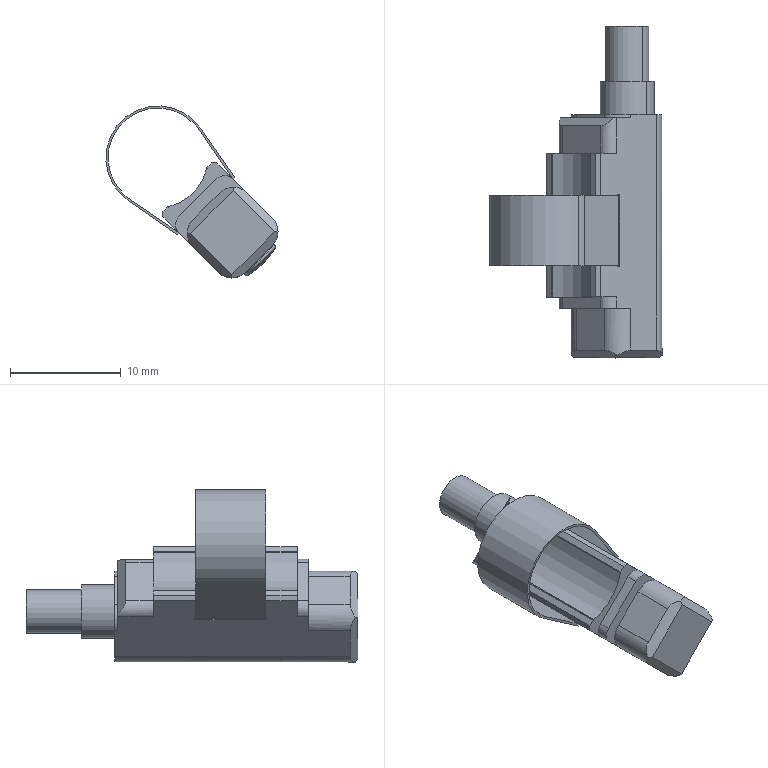Component | SolidWorks | MI-8x60-S-U-M-2(0)-1_CS1-M-S8-1 | 1 solid | 68 faces | box 15.56 x 30 x 15.56 mm | volume 1336 mm3 | plane 41 | cylinder 23 | sphere 2 | torus 2 | commonest cylinder face diameters 3.4 x6 9 x4 2 x4 9.4 x3 3.8 x2 3.9 x2 4.9 x2
build123d program:
from build123d import *

# Parameters (mm, degrees)
BOSS_EXTRUDE1_DEPTH      = 3.175
BOSS_EXTRUDE1_DEPTH_BACK = 3.175
BOSS_EXTRUDE2_DEPTH      = 18.5
CUT_EXTRUDE1_2_DEPTH     = 4.5
CUT_EXTRUDE2_DEPTH       = 5.5
CUT_EXTRUDE3_DEPTH       = 18.5
BOSS_EXTRUDE3_DEPTH      = 3.5
CUT_EXTRUDE4_DEPTH       = 3.25
CUT_EXTRUDE4_DEPTH_BACK  = 3.25
SKETCH7_W                = 7.3
SKETCH7_H                = 0.3
SKETCH8_R                = 2.45
BOSS_EXTRUDE4_DEPTH      = 25
SKETCH9_R                = 1.95
BOSS_EXTRUDE5_DEPTH      = 30
BOSS_EXTRUDE6_DEPTH      = 3.2
CUT_EXTRUDE5_DEPTH       = 5
CUT_EXTRUDE5_DEPTH_BACK  = 5
CUT_EXTRUDE6_DEPTH       = 5
CUT_EXTRUDE6_DEPTH_BACK  = 5
CUT_EXTRUDE7_DEPTH       = 10
CUT_EXTRUDE7_DEPTH_BACK  = 10
SKETCH1_R                = 4.5
CUT_EXTRUDE1_DEPTH       = 100


with BuildPart() as part:
    # Sketch1_2 → Boss-Extrude1 (new, two sides: drawn at the far end of the back side and taken through both)
    with BuildSketch(Plane(origin=(11.5, 0, 0), x_dir=(0, 0, -1), z_dir=(1, 0, 0)).offset(-BOSS_EXTRUDE1_DEPTH_BACK)):
        with BuildLine():
            Line((4.624, 0.8406), (3.65, 6.2))
            Line((3.65, 6.2), (-3.65, 6.2))
            Line((-3.65, 6.2), (-4.624, 0.8406))
            ThreePointArc((-4.624, 0.8406), (0, -4.7), (4.624, 0.8406))
        make_face()
        with BuildLine():
            Line((4.422, 0.8321), (3.45, 6))
            Line((3.45, 6), (-3.45, 6))
            Line((-3.45, 6), (-4.422, 0.8321))
            ThreePointArc((-4.422, 0.8321), (0, -4.5), (4.422, 0.8321))
        make_face(mode=Mode.SUBTRACT)
    extrude(amount=BOSS_EXTRUDE1_DEPTH + BOSS_EXTRUDE1_DEPTH_BACK)

    # Sketch2 → Boss-Extrude2 (add)
    with BuildSketch(Plane(origin=(0, 0, 0), x_dir=(0, 0, -1), z_dir=(1, 0, 0))):
        with BuildLine():
            Line((-3.45, 4.095), (-3.096, 3.742))
            Line((-3.096, 3.742), (-2.5, 3.742))
            Line((-2.5, 3.742), (-2.5, 3.8))
            Line((-2.5, 3.8), (2.5, 3.8))
            Line((2.5, 3.8), (2.5, 3.742))
            Line((2.5, 3.742), (3.096, 3.742))
            Line((3.096, 3.742), (3.45, 4.095))
            Line((3.45, 4.095), (3.45, 11.2))
            ThreePointArc((3.45, 11.2), (2.952, 12.402), (1.75, 12.9))
            Line((1.75, 12.9), (-1.75, 12.9))
            ThreePointArc((-1.75, 12.9), (-2.952, 12.402), (-3.45, 11.2))
            Line((-3.45, 11.2), (-3.45, 4.095))
        make_face()
    extrude(amount=BOSS_EXTRUDE2_DEPTH)

    # Sketch3 → Cut-Extrude1_2 (cut)
    with BuildSketch(Plane(origin=(0, 0, 0), x_dir=(0, 0, -1), z_dir=(1, 0, 0))):
        with BuildLine():
            Line((-3.45, 4.095), (-3.096, 3.742))
            Line((-3.096, 3.742), (-2.5, 3.742))
            Line((-2.5, 3.742), (-2.5, 3.8))
            Line((-2.5, 3.8), (2.5, 3.8))
            Line((2.5, 3.8), (2.5, 3.742))
            Line((2.5, 3.742), (3.096, 3.742))
            Line((3.096, 3.742), (3.45, 4.095))
            Line((3.45, 4.095), (3.45, 7.9))
            ThreePointArc((3.45, 7.9), (2.952, 6.698), (1.75, 6.2))
            Line((1.75, 6.2), (-1.75, 6.2))
            ThreePointArc((-1.75, 6.2), (-2.952, 6.698), (-3.45, 7.9))
            Line((-3.45, 7.9), (-3.45, 4.095))
        make_face()
    extrude(amount=CUT_EXTRUDE1_2_DEPTH, mode=Mode.SUBTRACT)

    # Sketch4 → Cut-Extrude2 (cut)
    with BuildSketch(Plane(origin=(0, 0, 0), x_dir=(0, 0, -1), z_dir=(1, 0, 0))):
        with BuildLine():
            Line((-3.45, 4.095), (-3.096, 3.742))
            Line((-3.096, 3.742), (-2.5, 3.742))
            Line((-2.5, 3.742), (-2.5, 3.8))
            Line((-2.5, 3.8), (2.5, 3.8))
            Line((2.5, 3.8), (2.5, 3.742))
            Line((2.5, 3.742), (3.096, 3.742))
            Line((3.096, 3.742), (3.45, 4.095))
            Line((3.45, 4.095), (3.45, 6.1))
            ThreePointArc((3.45, 6.1), (3.157, 5.393), (2.45, 5.1))
            Line((2.45, 5.1), (-2.45, 5.1))
            ThreePointArc((-2.45, 5.1), (-3.157, 5.393), (-3.45, 6.1))
            Line((-3.45, 6.1), (-3.45, 4.095))
        make_face()
    extrude(amount=CUT_EXTRUDE2_DEPTH, mode=Mode.SUBTRACT)

    # Sketch5 → Cut-Extrude3 (cut)
    with BuildSketch(Plane(origin=(0, 0, 0), x_dir=(0, 0, -1), z_dir=(1, 0, 0))):
        with BuildLine():
            Line((-2.5, 3.742), (-2.5, 3.4))
            Line((-2.5, 3.4), (2.5, 3.4))
            Line((2.5, 3.4), (2.5, 3.742))
            Line((2.5, 3.742), (2.18, 3.742))
            ThreePointArc((2.18, 3.742), (0, 4.242), (-2.18, 3.742))
            Line((-2.18, 3.742), (-2.5, 3.742))
        make_face()
    extrude(amount=CUT_EXTRUDE3_DEPTH, mode=Mode.SUBTRACT)

    # Sketch6 → Boss-Extrude3 (add)
    with BuildSketch(Plane(origin=(18.5, 0, 0), x_dir=(0, 0, -1), z_dir=(1, 0, 0))):
        with BuildLine():
            Line((-3.45, 11.2), (-3.45, 7.9))
            ThreePointArc((-3.45, 7.9), (-2.952, 6.698), (-1.75, 6.2))
            Line((-1.75, 6.2), (1.75, 6.2))
            ThreePointArc((1.75, 6.2), (2.952, 6.698), (3.45, 7.9))
            Line((3.45, 7.9), (3.45, 11.2))
            ThreePointArc((3.45, 11.2), (2.952, 12.402), (1.75, 12.9))
            Line((1.75, 12.9), (-1.75, 12.9))
            ThreePointArc((-1.75, 12.9), (-2.952, 12.402), (-3.45, 11.2))
        make_face()
    extrude(amount=BOSS_EXTRUDE3_DEPTH)

    # Sketch7 → Cut-Extrude4 (cut, two sides: drawn at the far end of the back side and taken through both)
    with BuildSketch(Plane(origin=(11.5, 0, 0), x_dir=(0, 0, -1), z_dir=(1, 0, 0)).offset(-CUT_EXTRUDE4_DEPTH_BACK)):
        with Locations((0, 6.35)):
            Rectangle(SKETCH7_W, SKETCH7_H)
    extrude(amount=CUT_EXTRUDE4_DEPTH + CUT_EXTRUDE4_DEPTH_BACK, mode=Mode.SUBTRACT)

    # Sketch8 → Boss-Extrude4 (add)
    with BuildSketch(Plane(origin=(0, 0, 0), x_dir=(0, 0, -1), z_dir=(1, 0, 0))):
        with Locations((1, 9.9)):
            Circle(SKETCH8_R)
    extrude(amount=BOSS_EXTRUDE4_DEPTH)

    # Sketch9 → Boss-Extrude5 (add)
    with BuildSketch(Plane(origin=(0, 0, 0), x_dir=(0, 0, -1), z_dir=(1, 0, 0))):
        with Locations((1, 9.9)):
            Circle(SKETCH9_R)
    extrude(amount=BOSS_EXTRUDE5_DEPTH)

    # Sketch10 → Boss-Extrude6 (add)
    with BuildSketch(Plane(origin=(18.5, 0, 0), x_dir=(0, 0, -1), z_dir=(1, 0, 0))):
        with BuildLine():
            Line((-2.45, 5.1), (2.45, 5.1))
            ThreePointArc((2.45, 5.1), (3.157, 5.393), (3.45, 6.1))
            Line((3.45, 6.1), (3.45, 7.9))
            ThreePointArc((3.45, 7.9), (2.952, 6.698), (1.75, 6.2))
            Line((1.75, 6.2), (-1.75, 6.2))
            ThreePointArc((-1.75, 6.2), (-2.952, 6.698), (-3.45, 7.9))
            Line((-3.45, 7.9), (-3.45, 6.1))
            ThreePointArc((-3.45, 6.1), (-3.157, 5.393), (-2.45, 5.1))
        make_face()
    extrude(amount=BOSS_EXTRUDE6_DEPTH)

    # Sketch11 → Cut-Extrude5 (cut, two sides: drawn at the far end of the back side and taken through both)
    with BuildSketch(Plane.XY.offset(-CUT_EXTRUDE5_DEPTH_BACK)):
        Polygon((20.993, 5.1), (20.993, 4.1), (22.7, 4.1), (22.7, 5.807), (21.7, 5.807), align=None)
    extrude(amount=CUT_EXTRUDE5_DEPTH + CUT_EXTRUDE5_DEPTH_BACK, mode=Mode.SUBTRACT)

    # Sketch12 → Cut-Extrude6 (cut, two sides: drawn at the far end of the back side and taken through both)
    with BuildSketch(Plane.XY.offset(-CUT_EXTRUDE6_DEPTH_BACK)):
        Polygon((-1, 13.9), (-1, 5.2), (0.7071, 5.2), (0.7071, 6.2), (0, 6.907), (0, 12.193), (0.7071, 12.9), (0.7071, 13.9), align=None)
    extrude(amount=CUT_EXTRUDE6_DEPTH + CUT_EXTRUDE6_DEPTH_BACK, mode=Mode.SUBTRACT)

    # Sketch13 → Cut-Extrude7 (cut, two sides: drawn at the far end of the back side and taken through both)
    with BuildSketch(Plane(origin=(0, 12.9, 0), x_dir=(1, 0, 0), z_dir=(0, 1, 0)).offset(-CUT_EXTRUDE7_DEPTH_BACK)):
        Polygon((-1, -4.45), (0.7071, -4.45), (0.7071, -3.45), (0, -2.743), (0, 2.743), (0.7071, 3.45), (0.7071, 4.45), (-1, 4.45), align=None)
    extrude(amount=CUT_EXTRUDE7_DEPTH + CUT_EXTRUDE7_DEPTH_BACK, mode=Mode.SUBTRACT)

    # Sketch14 → Revolve1 (revolve)
    with BuildSketch(Plane(origin=(7.1, 0, 0), x_dir=(0, 0, -1), z_dir=(1, 0, 0)), mode=Mode.PRIVATE) as revolve1_sk:
        with BuildLine():
            Line((0, 12.9), (-1.9, 12.9))
            Line((-1.9, 12.9), (-1.9, 13.015))
            ThreePointArc((-1.9, 13.015), (-1.85, 13.166), (-1.72, 13.256))
            ThreePointArc((-1.72, 13.256), (-0.8685, 13.439), (0, 13.5))
            Line((0, 13.5), (0, 12.9))
        make_face()
    revolve(revolve1_sk.sketch.rotate(Axis((7.1, 13.5, 0), (0, -1, 0)), 180), axis=Axis((7.1, 13.5, 0), (0, -1, 0)))

    # Sketch1 → Cut-Extrude1 (cut, symmetric)
    with BuildSketch(Plane(origin=(0, 0, 0), x_dir=(0, 0, -1), z_dir=(1, 0, 0))):
        Circle(SKETCH1_R)
    extrude(amount=CUT_EXTRUDE1_DEPTH, both=True, mode=Mode.SUBTRACT)


solid = part.part

# Placed as in the assembly
solid = solid.moved(Location((-44.181, -31.688, -311.979), (-180, -45, -90)))